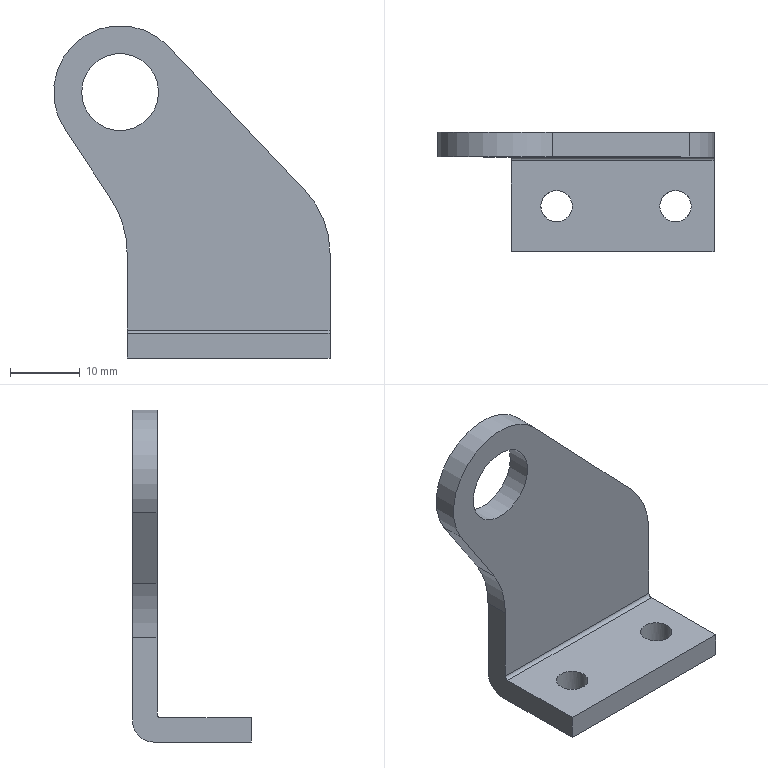Component | NX | RIGHT_SIDE_PLATE | 1 solid | 17 faces | volume 5118 mm3 | plane 9 | cylinder 8 | commonest cylinder face diameters 4.5 x2 28 x1 19 x1 26 x1 11 x1 1 x1 6 x1